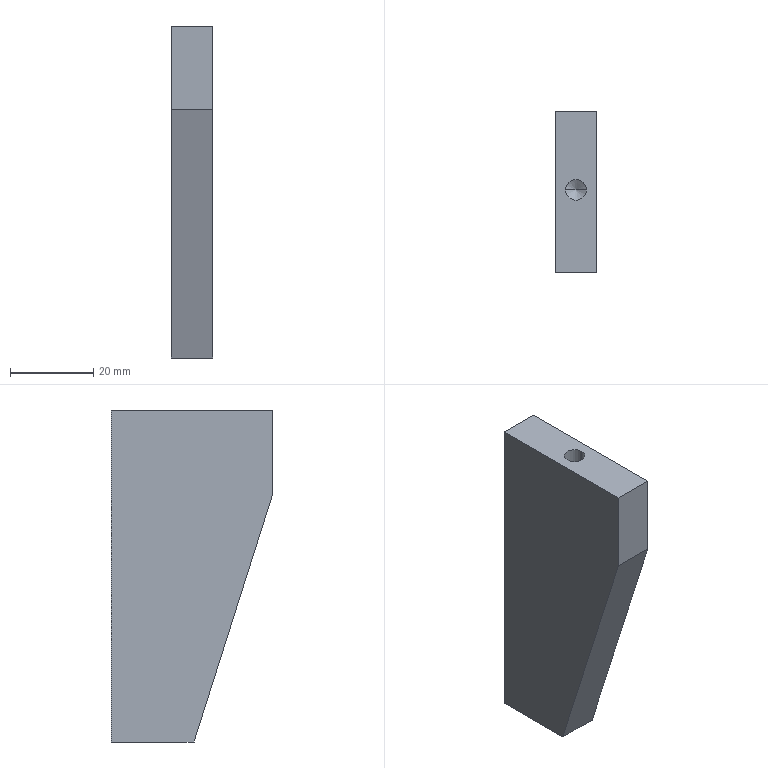Component | SolidWorks | 75-02-19StirringMotorSupportPlate-1 | 1 solid | 19 faces | box 10 x 39 x 80 mm | volume 24587 mm3 | plane 7 | cylinder 6 | cone 6 | commonest cylinder face diameters 5 x6 | material A3 Steel
build123d program:
from build123d import *

# Parameters (mm, degrees)
BOSS_EXTRUDE1_DEPTH   = 5
M6_TAPPED_HOLE1_D     = 5
M6_TAPPED_HOLE1_DEPTH = 15
M6_TAPPED_HOLE1_TIP   = 1.502
M6_TAPPED_HOLE2_D     = 5
M6_TAPPED_HOLE2_DEPTH = 15
M6_TAPPED_HOLE2_TIP   = 1.502


with BuildPart() as part:
    # Sketch1 → Boss-Extrude1 (new, symmetric)
    with BuildSketch(Plane.XY):
        Polygon((0, 39), (0, 0), (80, 0), (80, 20), (20, 39), align=None)
    extrude(amount=BOSS_EXTRUDE1_DEPTH, both=True)

    # M6 Tapped Hole1
    with Locations(Plane(origin=(60, 0, 0), x_dir=(0, 0, -1), z_dir=(0, -1, 0))):
        with Locations((0, 0), (0, -40)):
            Hole(M6_TAPPED_HOLE1_D / 2, depth=M6_TAPPED_HOLE1_DEPTH)
            with Locations((0, 0, -(M6_TAPPED_HOLE1_DEPTH + M6_TAPPED_HOLE1_TIP / 2))):  # 118° drill point
                Cone(0, M6_TAPPED_HOLE1_D / 2, M6_TAPPED_HOLE1_TIP, mode=Mode.SUBTRACT)

    # M6 Tapped Hole2
    with Locations(Plane(origin=(0, 19, 0), x_dir=(0, -1, 0), z_dir=(-1, 0, 0))):
        with Locations((0, 0)):
            Hole(M6_TAPPED_HOLE2_D / 2, depth=M6_TAPPED_HOLE2_DEPTH)
            with Locations((0, 0, -(M6_TAPPED_HOLE2_DEPTH + M6_TAPPED_HOLE2_TIP / 2))):  # 118° drill point
                Cone(0, M6_TAPPED_HOLE2_D / 2, M6_TAPPED_HOLE2_TIP, mode=Mode.SUBTRACT)


solid = part.part

# Placed as in the assembly
solid = solid.moved(Location((22.2, 105.857, 2.75), (180, -90, 0)))
STEP:
#1=COLOUR_RGB('',0.7922,0.8196,0.9333);
#2=FILL_AREA_STYLE_COLOUR('',#1);
#3=FILL_AREA_STYLE('',(#2));
#4=SURFACE_STYLE_FILL_AREA(#3);
#5=SURFACE_SIDE_STYLE('',(#4));
#6=SURFACE_STYLE_USAGE(.BOTH.,#5);
#7=PRESENTATION_STYLE_ASSIGNMENT((#6));
#8=CARTESIAN_POINT('',(0.9724,3.42,-0.4823));
#9=VERTEX_POINT('',#8);
#10=CARTESIAN_POINT('',(0.7756,3.42,-0.4823));
#11=VERTEX_POINT('',#10);
#12=CARTESIAN_POINT('',(0.874,3.42,-0.4823));
#13=DIRECTION('',(0.,-0.,1.));
#14=DIRECTION('',(-1.,0.,0.));
#15=AXIS2_PLACEMENT_3D('',#12,#13,#14);
#16=CIRCLE('',#15,0.09843);
#17=EDGE_CURVE('',#9,#11,#16,.T.);
#18=ORIENTED_EDGE('',*,*,#17,.F.);
#19=CARTESIAN_POINT('',(0.9724,3.42,0.1083));
#20=VERTEX_POINT('',#19);
#21=CARTESIAN_POINT('',(0.9724,3.42,0.1083));
#22=DIRECTION('',(0.,-0.,1.));
#23=VECTOR('',#22,39.37);
#24=LINE('',#21,#23);
#25=EDGE_CURVE('',#9,#20,#24,.T.);
#26=ORIENTED_EDGE('',*,*,#25,.T.);
#27=CARTESIAN_POINT('',(0.7756,3.42,0.1083));
#28=VERTEX_POINT('',#27);
#29=CARTESIAN_POINT('',(0.874,3.42,0.1083));
#30=DIRECTION('',(0.,-0.,1.));
#31=DIRECTION('',(-1.,0.,0.));
#32=AXIS2_PLACEMENT_3D('',#29,#30,#31);
#33=CIRCLE('',#32,0.09843);
#34=EDGE_CURVE('',#20,#28,#33,.T.);
#35=ORIENTED_EDGE('',*,*,#34,.T.);
#36=CARTESIAN_POINT('',(0.7756,3.42,0.1083));
#37=DIRECTION('',(0.,-0.,1.));
#38=VECTOR('',#37,39.37);
#39=LINE('',#36,#38);
#40=EDGE_CURVE('',#11,#28,#39,.T.);
#41=ORIENTED_EDGE('',*,*,#40,.F.);
#42=EDGE_LOOP('',(#18,#26,#35,#41));
#43=FACE_OUTER_BOUND('',#42,.T.);
#44=CARTESIAN_POINT('',(0.874,3.42,0.1083));
#45=DIRECTION('',(0.,-0.,1.));
#46=DIRECTION('',(-1.,0.,0.));
#47=AXIS2_PLACEMENT_3D('',#44,#45,#46);
#48=CYLINDRICAL_SURFACE('',#47,0.09843);
#49=ADVANCED_FACE('',(#43),#48,.F.);
#50=CARTESIAN_POINT('',(0.874,3.42,-0.5414));
#51=VERTEX_POINT('',#50);
#52=CARTESIAN_POINT('',(0.7756,3.42,-0.4823));
#53=DIRECTION('',(-0.8572,0.,0.515));
#54=VECTOR('',#53,39.37);
#55=LINE('',#52,#54);
#56=EDGE_CURVE('',#51,#11,#55,.T.);
#57=ORIENTED_EDGE('',*,*,#56,.F.);
#58=CARTESIAN_POINT('',(0.9724,3.42,-0.4823));
#59=DIRECTION('',(0.8572,-0.,0.515));
#60=VECTOR('',#59,39.37);
#61=LINE('',#58,#60);
#62=EDGE_CURVE('',#51,#9,#61,.T.);
#63=ORIENTED_EDGE('',*,*,#62,.T.);
#64=ORIENTED_EDGE('',*,*,#17,.T.);
#65=EDGE_LOOP('',(#57,#63,#64));
#66=FACE_OUTER_BOUND('',#65,.T.);
#67=CARTESIAN_POINT('',(0.874,3.42,-0.4823));
#68=DIRECTION('',(0.,-0.,1.));
#69=DIRECTION('',(-1.,0.,0.));
#70=AXIS2_PLACEMENT_3D('',#67,#68,#69);
#71=CONICAL_SURFACE('',#70,0.09843,1.03);
#72=ADVANCED_FACE('',(#66),#71,.F.);
#73=CARTESIAN_POINT('',(0.7756,3.577,-2.254));
#74=VERTEX_POINT('',#73);
#75=CARTESIAN_POINT('',(0.9724,3.577,-2.254));
#76=VERTEX_POINT('',#75);
#77=CARTESIAN_POINT('',(0.874,3.577,-2.254));
#78=DIRECTION('',(0.,1.,0.));
#79=DIRECTION('',(1.,0.,0.));
#80=AXIS2_PLACEMENT_3D('',#77,#78,#79);
#81=CIRCLE('',#80,0.09843);
#82=EDGE_CURVE('',#74,#76,#81,.T.);
#83=ORIENTED_EDGE('',*,*,#82,.F.);
#84=CARTESIAN_POINT('',(0.7756,4.168,-2.254));
#85=VERTEX_POINT('',#84);
#86=CARTESIAN_POINT('',(0.7756,4.168,-2.254));
#87=DIRECTION('',(0.,1.,0.));
#88=VECTOR('',#87,39.37);
#89=LINE('',#86,#88);
#90=EDGE_CURVE('',#74,#85,#89,.T.);
#91=ORIENTED_EDGE('',*,*,#90,.T.);
#92=CARTESIAN_POINT('',(0.9724,4.168,-2.254));
#93=VERTEX_POINT('',#92);
#94=CARTESIAN_POINT('',(0.874,4.168,-2.254));
#95=DIRECTION('',(0.,1.,0.));
#96=DIRECTION('',(1.,0.,0.));
#97=AXIS2_PLACEMENT_3D('',#94,#95,#96);
#98=CIRCLE('',#97,0.09843);
#99=EDGE_CURVE('',#85,#93,#98,.T.);
#100=ORIENTED_EDGE('',*,*,#99,.T.);
#101=CARTESIAN_POINT('',(0.9724,4.168,-2.254));
#102=DIRECTION('',(0.,1.,0.));
#103=VECTOR('',#102,39.37);
#104=LINE('',#101,#103);
#105=EDGE_CURVE('',#76,#93,#104,.T.);
#106=ORIENTED_EDGE('',*,*,#105,.F.);
#107=EDGE_LOOP('',(#83,#91,#100,#106));
#108=FACE_OUTER_BOUND('',#107,.T.);
#109=CARTESIAN_POINT('',(0.874,4.168,-2.254));
#110=DIRECTION('',(0.,1.,0.));
#111=DIRECTION('',(1.,0.,0.));
#112=AXIS2_PLACEMENT_3D('',#109,#110,#111);
#113=CYLINDRICAL_SURFACE('',#112,0.09843);
#114=ADVANCED_FACE('',(#108),#113,.F.);
#115=CARTESIAN_POINT('',(0.874,3.518,-2.254));
#116=VERTEX_POINT('',#115);
#117=CARTESIAN_POINT('',(0.9724,3.577,-2.254));
#118=DIRECTION('',(0.8572,0.515,-0.));
#119=VECTOR('',#118,39.37);
#120=LINE('',#117,#119);
#121=EDGE_CURVE('',#116,#76,#120,.T.);
#122=ORIENTED_EDGE('',*,*,#121,.F.);
#123=CARTESIAN_POINT('',(0.7756,3.577,-2.254));
#124=DIRECTION('',(-0.8572,0.515,0.));
#125=VECTOR('',#124,39.37);
#126=LINE('',#123,#125);
#127=EDGE_CURVE('',#116,#74,#126,.T.);
#128=ORIENTED_EDGE('',*,*,#127,.T.);
#129=ORIENTED_EDGE('',*,*,#82,.T.);
#130=EDGE_LOOP('',(#122,#128,#129));
#131=FACE_OUTER_BOUND('',#130,.T.);
#132=CARTESIAN_POINT('',(0.874,3.577,-2.254));
#133=DIRECTION('',(0.,1.,0.));
#134=DIRECTION('',(1.,0.,0.));
#135=AXIS2_PLACEMENT_3D('',#132,#133,#134);
#136=CONICAL_SURFACE('',#135,0.09843,1.03);
#137=ADVANCED_FACE('',(#131),#136,.F.);
#138=CARTESIAN_POINT('',(0.7756,3.577,-0.6791));
#139=VERTEX_POINT('',#138);
#140=CARTESIAN_POINT('',(0.9724,3.577,-0.6791));
#141=VERTEX_POINT('',#140);
#142=CARTESIAN_POINT('',(0.874,3.577,-0.6791));
#143=DIRECTION('',(0.,1.,0.));
#144=DIRECTION('',(1.,0.,0.));
#145=AXIS2_PLACEMENT_3D('',#142,#143,#144);
#146=CIRCLE('',#145,0.09843);
#147=EDGE_CURVE('',#139,#141,#146,.T.);
#148=ORIENTED_EDGE('',*,*,#147,.F.);
#149=CARTESIAN_POINT('',(0.7756,4.168,-0.6791));
#150=VERTEX_POINT('',#149);
#151=CARTESIAN_POINT('',(0.7756,4.168,-0.6791));
#152=DIRECTION('',(0.,1.,0.));
#153=VECTOR('',#152,39.37);
#154=LINE('',#151,#153);
#155=EDGE_CURVE('',#139,#150,#154,.T.);
#156=ORIENTED_EDGE('',*,*,#155,.T.);
#157=CARTESIAN_POINT('',(0.9724,4.168,-0.6791));
#158=VERTEX_POINT('',#157);
#159=CARTESIAN_POINT('',(0.874,4.168,-0.6791));
#160=DIRECTION('',(0.,1.,0.));
#161=DIRECTION('',(1.,0.,0.));
#162=AXIS2_PLACEMENT_3D('',#159,#160,#161);
#163=CIRCLE('',#162,0.09843);
#164=EDGE_CURVE('',#150,#158,#163,.T.);
#165=ORIENTED_EDGE('',*,*,#164,.T.);
#166=CARTESIAN_POINT('',(0.9724,4.168,-0.6791));
#167=DIRECTION('',(0.,1.,0.));
#168=VECTOR('',#167,39.37);
#169=LINE('',#166,#168);
#170=EDGE_CURVE('',#141,#158,#169,.T.);
#171=ORIENTED_EDGE('',*,*,#170,.F.);
#172=EDGE_LOOP('',(#148,#156,#165,#171));
#173=FACE_OUTER_BOUND('',#172,.T.);
#174=CARTESIAN_POINT('',(0.874,4.168,-0.6791));
#175=DIRECTION('',(0.,1.,0.));
#176=DIRECTION('',(1.,0.,0.));
#177=AXIS2_PLACEMENT_3D('',#174,#175,#176);
#178=CYLINDRICAL_SURFACE('',#177,0.09843);
#179=ADVANCED_FACE('',(#173),#178,.F.);
#180=CARTESIAN_POINT('',(0.874,3.518,-0.6791));
#181=VERTEX_POINT('',#180);
#182=CARTESIAN_POINT('',(0.9724,3.577,-0.6791));
#183=DIRECTION('',(0.8572,0.515,-0.));
#184=VECTOR('',#183,39.37);
#185=LINE('',#182,#184);
#186=EDGE_CURVE('',#181,#141,#185,.T.);
#187=ORIENTED_EDGE('',*,*,#186,.F.);
#188=CARTESIAN_POINT('',(0.7756,3.577,-0.6791));
#189=DIRECTION('',(-0.8572,0.515,0.));
#190=VECTOR('',#189,39.37);
#191=LINE('',#188,#190);
#192=EDGE_CURVE('',#181,#139,#191,.T.);
#193=ORIENTED_EDGE('',*,*,#192,.T.);
#194=ORIENTED_EDGE('',*,*,#147,.T.);
#195=EDGE_LOOP('',(#187,#193,#194));
#196=FACE_OUTER_BOUND('',#195,.T.);
#197=CARTESIAN_POINT('',(0.874,3.577,-0.6791));
#198=DIRECTION('',(0.,1.,0.));
#199=DIRECTION('',(1.,0.,0.));
#200=AXIS2_PLACEMENT_3D('',#197,#198,#199);
#201=CONICAL_SURFACE('',#200,0.09843,1.03);
#202=ADVANCED_FACE('',(#196),#201,.F.);
#203=CARTESIAN_POINT('',(1.071,2.632,-0.6791));
#204=VERTEX_POINT('',#203);
#205=CARTESIAN_POINT('',(1.071,2.632,0.1083));
#206=VERTEX_POINT('',#205);
#207=CARTESIAN_POINT('',(1.071,2.632,-0.6791));
#208=DIRECTION('',(0.,-0.,1.));
#209=VECTOR('',#208,39.37);
#210=LINE('',#207,#209);
#211=EDGE_CURVE('',#204,#206,#210,.T.);
#212=ORIENTED_EDGE('',*,*,#211,.T.);
#213=CARTESIAN_POINT('',(0.6772,2.632,0.1083));
#214=VERTEX_POINT('',#213);
#215=CARTESIAN_POINT('',(0.6772,2.632,0.1083));
#216=DIRECTION('',(1.,-0.,-0.));
#217=VECTOR('',#216,39.37);
#218=LINE('',#215,#217);
#219=EDGE_CURVE('',#214,#206,#218,.T.);
#220=ORIENTED_EDGE('',*,*,#219,.F.);
#221=CARTESIAN_POINT('',(0.6772,2.632,-0.6791));
#222=VERTEX_POINT('',#221);
#223=CARTESIAN_POINT('',(0.6772,2.632,-0.6791));
#224=DIRECTION('',(0.,-0.,1.));
#225=VECTOR('',#224,39.37);
#226=LINE('',#223,#225);
#227=EDGE_CURVE('',#222,#214,#226,.T.);
#228=ORIENTED_EDGE('',*,*,#227,.F.);
#229=CARTESIAN_POINT('',(0.6772,2.632,-0.6791));
#230=DIRECTION('',(1.,-0.,-0.));
#231=VECTOR('',#230,39.37);
#232=LINE('',#229,#231);
#233=EDGE_CURVE('',#222,#204,#232,.T.);
#234=ORIENTED_EDGE('',*,*,#233,.T.);
#235=EDGE_LOOP('',(#212,#220,#228,#234));
#236=FACE_OUTER_BOUND('',#235,.T.);
#237=CARTESIAN_POINT('',(0.6772,2.632,-0.6791));
#238=DIRECTION('',(0.,1.,0.));
#239=DIRECTION('',(1.,-0.,-0.));
#240=AXIS2_PLACEMENT_3D('',#237,#238,#239);
#241=PLANE('',#240);
#242=ADVANCED_FACE('',(#236),#241,.F.);
#243=CARTESIAN_POINT('',(0.874,3.42,0.1083));
#244=DIRECTION('',(0.,-0.,1.));
#245=DIRECTION('',(-1.,0.,0.));
#246=AXIS2_PLACEMENT_3D('',#243,#244,#245);
#247=CIRCLE('',#246,0.09843);
#248=EDGE_CURVE('',#28,#20,#247,.T.);
#249=ORIENTED_EDGE('',*,*,#248,.F.);
#250=ORIENTED_EDGE('',*,*,#34,.F.);
#251=EDGE_LOOP('',(#249,#250));
#252=FACE_BOUND('',#251,.T.);
#253=CARTESIAN_POINT('',(1.071,4.168,0.1083));
#254=VERTEX_POINT('',#253);
#255=CARTESIAN_POINT('',(1.071,2.632,0.1083));
#256=DIRECTION('',(0.,1.,0.));
#257=VECTOR('',#256,39.37);
#258=LINE('',#255,#257);
#259=EDGE_CURVE('',#206,#254,#258,.T.);
#260=ORIENTED_EDGE('',*,*,#259,.T.);
#261=CARTESIAN_POINT('',(0.6772,4.168,0.1083));
#262=VERTEX_POINT('',#261);
#263=CARTESIAN_POINT('',(0.6772,4.168,0.1083));
#264=DIRECTION('',(1.,-0.,-0.));
#265=VECTOR('',#264,39.37);
#266=LINE('',#263,#265);
#267=EDGE_CURVE('',#262,#254,#266,.T.);
#268=ORIENTED_EDGE('',*,*,#267,.F.);
#269=CARTESIAN_POINT('',(0.6772,2.632,0.1083));
#270=DIRECTION('',(0.,1.,0.));
#271=VECTOR('',#270,39.37);
#272=LINE('',#269,#271);
#273=EDGE_CURVE('',#214,#262,#272,.T.);
#274=ORIENTED_EDGE('',*,*,#273,.F.);
#275=ORIENTED_EDGE('',*,*,#219,.T.);
#276=EDGE_LOOP('',(#260,#268,#274,#275));
#277=FACE_OUTER_BOUND('',#276,.T.);
#278=CARTESIAN_POINT('',(0.6772,2.632,0.1083));
#279=DIRECTION('',(-0.,0.,-1.));
#280=DIRECTION('',(-0.,-1.,-0.));
#281=AXIS2_PLACEMENT_3D('',#278,#279,#280);
#282=PLANE('',#281);
#283=ADVANCED_FACE('',(#252,#277),#282,.F.);
#284=CARTESIAN_POINT('',(0.874,4.168,-2.254));
#285=DIRECTION('',(0.,1.,0.));
#286=DIRECTION('',(1.,0.,0.));
#287=AXIS2_PLACEMENT_3D('',#284,#285,#286);
#288=CIRCLE('',#287,0.09843);
#289=EDGE_CURVE('',#93,#85,#288,.T.);
#290=ORIENTED_EDGE('',*,*,#289,.F.);
#291=ORIENTED_EDGE('',*,*,#99,.F.);
#292=EDGE_LOOP('',(#290,#291));
#293=FACE_BOUND('',#292,.T.);
#294=CARTESIAN_POINT('',(0.874,4.168,-0.6791));
#295=DIRECTION('',(0.,1.,0.));
#296=DIRECTION('',(1.,0.,0.));
#297=AXIS2_PLACEMENT_3D('',#294,#295,#296);
#298=CIRCLE('',#297,0.09843);
#299=EDGE_CURVE('',#158,#150,#298,.T.);
#300=ORIENTED_EDGE('',*,*,#299,.F.);
#301=ORIENTED_EDGE('',*,*,#164,.F.);
#302=EDGE_LOOP('',(#300,#301));
#303=FACE_BOUND('',#302,.T.);
#304=CARTESIAN_POINT('',(1.071,4.168,-3.041));
#305=VERTEX_POINT('',#304);
#306=CARTESIAN_POINT('',(1.071,4.168,0.1083));
#307=DIRECTION('',(-0.,0.,-1.));
#308=VECTOR('',#307,39.37);
#309=LINE('',#306,#308);
#310=EDGE_CURVE('',#254,#305,#309,.T.);
#311=ORIENTED_EDGE('',*,*,#310,.T.);
#312=CARTESIAN_POINT('',(0.6772,4.168,-3.041));
#313=VERTEX_POINT('',#312);
#314=CARTESIAN_POINT('',(0.6772,4.168,-3.041));
#315=DIRECTION('',(1.,-0.,-0.));
#316=VECTOR('',#315,39.37);
#317=LINE('',#314,#316);
#318=EDGE_CURVE('',#313,#305,#317,.T.);
#319=ORIENTED_EDGE('',*,*,#318,.F.);
#320=CARTESIAN_POINT('',(0.6772,4.168,0.1083));
#321=DIRECTION('',(-0.,0.,-1.));
#322=VECTOR('',#321,39.37);
#323=LINE('',#320,#322);
#324=EDGE_CURVE('',#262,#313,#323,.T.);
#325=ORIENTED_EDGE('',*,*,#324,.F.);
#326=ORIENTED_EDGE('',*,*,#267,.T.);
#327=EDGE_LOOP('',(#311,#319,#325,#326));
#328=FACE_OUTER_BOUND('',#327,.T.);
#329=CARTESIAN_POINT('',(0.6772,4.168,0.1083));
#330=DIRECTION('',(-0.,-1.,-0.));
#331=DIRECTION('',(-1.,0.,0.));
#332=AXIS2_PLACEMENT_3D('',#329,#330,#331);
#333=PLANE('',#332);
#334=ADVANCED_FACE('',(#293,#303,#328),#333,.F.);
#335=CARTESIAN_POINT('',(1.071,3.38,-3.041));
#336=VERTEX_POINT('',#335);
#337=CARTESIAN_POINT('',(1.071,4.168,-3.041));
#338=DIRECTION('',(-0.,-1.,-0.));
#339=VECTOR('',#338,39.37);
#340=LINE('',#337,#339);
#341=EDGE_CURVE('',#305,#336,#340,.T.);
#342=ORIENTED_EDGE('',*,*,#341,.T.);
#343=CARTESIAN_POINT('',(0.6772,3.38,-3.041));
#344=VERTEX_POINT('',#343);
#345=CARTESIAN_POINT('',(0.6772,3.38,-3.041));
#346=DIRECTION('',(1.,-0.,-0.));
#347=VECTOR('',#346,39.37);
#348=LINE('',#345,#347);
#349=EDGE_CURVE('',#344,#336,#348,.T.);
#350=ORIENTED_EDGE('',*,*,#349,.F.);
#351=CARTESIAN_POINT('',(0.6772,4.168,-3.041));
#352=DIRECTION('',(-0.,-1.,-0.));
#353=VECTOR('',#352,39.37);
#354=LINE('',#351,#353);
#355=EDGE_CURVE('',#313,#344,#354,.T.);
#356=ORIENTED_EDGE('',*,*,#355,.F.);
#357=ORIENTED_EDGE('',*,*,#318,.T.);
#358=EDGE_LOOP('',(#342,#350,#356,#357));
#359=FACE_OUTER_BOUND('',#358,.T.);
#360=CARTESIAN_POINT('',(0.6772,4.168,-3.041));
#361=DIRECTION('',(0.,-0.,1.));
#362=DIRECTION('',(-1.,0.,0.));
#363=AXIS2_PLACEMENT_3D('',#360,#361,#362);
#364=PLANE('',#363);
#365=ADVANCED_FACE('',(#359),#364,.F.);
#366=CARTESIAN_POINT('',(1.071,3.38,-3.041));
#367=DIRECTION('',(0.,-0.3019,0.9533));
#368=VECTOR('',#367,39.37);
#369=LINE('',#366,#368);
#370=EDGE_CURVE('',#336,#204,#369,.T.);
#371=ORIENTED_EDGE('',*,*,#370,.T.);
#372=ORIENTED_EDGE('',*,*,#233,.F.);
#373=CARTESIAN_POINT('',(0.6772,3.38,-3.041));
#374=DIRECTION('',(0.,-0.3019,0.9533));
#375=VECTOR('',#374,39.37);
#376=LINE('',#373,#375);
#377=EDGE_CURVE('',#344,#222,#376,.T.);
#378=ORIENTED_EDGE('',*,*,#377,.F.);
#379=ORIENTED_EDGE('',*,*,#349,.T.);
#380=EDGE_LOOP('',(#371,#372,#378,#379));
#381=FACE_OUTER_BOUND('',#380,.T.);
#382=CARTESIAN_POINT('',(0.6772,3.38,-3.041));
#383=DIRECTION('',(0.,0.9533,0.3019));
#384=DIRECTION('',(-0.,0.3019,-0.9533));
#385=AXIS2_PLACEMENT_3D('',#382,#383,#384);
#386=PLANE('',#385);
#387=ADVANCED_FACE('',(#381),#386,.F.);
#388=ORIENTED_EDGE('',*,*,#227,.T.);
#389=ORIENTED_EDGE('',*,*,#273,.T.);
#390=ORIENTED_EDGE('',*,*,#324,.T.);
#391=ORIENTED_EDGE('',*,*,#355,.T.);
#392=ORIENTED_EDGE('',*,*,#377,.T.);
#393=EDGE_LOOP('',(#388,#389,#390,#391,#392));
#394=FACE_OUTER_BOUND('',#393,.T.);
#395=CARTESIAN_POINT('',(0.6772,4.168,0.1083));
#396=DIRECTION('',(-1.,0.,0.));
#397=DIRECTION('',(-0.,0.,-1.));
#398=AXIS2_PLACEMENT_3D('',#395,#396,#397);
#399=PLANE('',#398);
#400=ADVANCED_FACE('',(#394),#399,.T.);
#401=ORIENTED_EDGE('',*,*,#211,.F.);
#402=ORIENTED_EDGE('',*,*,#370,.F.);
#403=ORIENTED_EDGE('',*,*,#341,.F.);
#404=ORIENTED_EDGE('',*,*,#310,.F.);
#405=ORIENTED_EDGE('',*,*,#259,.F.);
#406=EDGE_LOOP('',(#401,#402,#403,#404,#405));
#407=FACE_OUTER_BOUND('',#406,.T.);
#408=CARTESIAN_POINT('',(1.071,4.168,0.1083));
#409=DIRECTION('',(-1.,0.,0.));
#410=DIRECTION('',(-0.,0.,-1.));
#411=AXIS2_PLACEMENT_3D('',#408,#409,#410);
#412=PLANE('',#411);
#413=ADVANCED_FACE('',(#407),#412,.F.);
#414=ORIENTED_EDGE('',*,*,#192,.F.);
#415=ORIENTED_EDGE('',*,*,#186,.T.);
#416=CARTESIAN_POINT('',(0.874,3.577,-0.6791));
#417=DIRECTION('',(0.,1.,0.));
#418=DIRECTION('',(1.,0.,0.));
#419=AXIS2_PLACEMENT_3D('',#416,#417,#418);
#420=CIRCLE('',#419,0.09843);
#421=EDGE_CURVE('',#141,#139,#420,.T.);
#422=ORIENTED_EDGE('',*,*,#421,.T.);
#423=EDGE_LOOP('',(#414,#415,#422));
#424=FACE_OUTER_BOUND('',#423,.T.);
#425=CARTESIAN_POINT('',(0.874,3.577,-0.6791));
#426=DIRECTION('',(0.,1.,0.));
#427=DIRECTION('',(1.,0.,0.));
#428=AXIS2_PLACEMENT_3D('',#425,#426,#427);
#429=CONICAL_SURFACE('',#428,0.09843,1.03);
#430=ADVANCED_FACE('',(#424),#429,.F.);
#431=ORIENTED_EDGE('',*,*,#155,.F.);
#432=ORIENTED_EDGE('',*,*,#421,.F.);
#433=ORIENTED_EDGE('',*,*,#170,.T.);
#434=ORIENTED_EDGE('',*,*,#299,.T.);
#435=EDGE_LOOP('',(#431,#432,#433,#434));
#436=FACE_OUTER_BOUND('',#435,.T.);
#437=CARTESIAN_POINT('',(0.874,4.168,-0.6791));
#438=DIRECTION('',(0.,1.,0.));
#439=DIRECTION('',(1.,0.,0.));
#440=AXIS2_PLACEMENT_3D('',#437,#438,#439);
#441=CYLINDRICAL_SURFACE('',#440,0.09843);
#442=ADVANCED_FACE('',(#436),#441,.F.);
#443=ORIENTED_EDGE('',*,*,#127,.F.);
#444=ORIENTED_EDGE('',*,*,#121,.T.);
#445=CARTESIAN_POINT('',(0.874,3.577,-2.254));
#446=DIRECTION('',(0.,1.,0.));
#447=DIRECTION('',(1.,0.,0.));
#448=AXIS2_PLACEMENT_3D('',#445,#446,#447);
#449=CIRCLE('',#448,0.09843);
#450=EDGE_CURVE('',#76,#74,#449,.T.);
#451=ORIENTED_EDGE('',*,*,#450,.T.);
#452=EDGE_LOOP('',(#443,#444,#451));
#453=FACE_OUTER_BOUND('',#452,.T.);
#454=CARTESIAN_POINT('',(0.874,3.577,-2.254));
#455=DIRECTION('',(0.,1.,0.));
#456=DIRECTION('',(1.,0.,0.));
#457=AXIS2_PLACEMENT_3D('',#454,#455,#456);
#458=CONICAL_SURFACE('',#457,0.09843,1.03);
#459=ADVANCED_FACE('',(#453),#458,.F.);
#460=ORIENTED_EDGE('',*,*,#90,.F.);
#461=ORIENTED_EDGE('',*,*,#450,.F.);
#462=ORIENTED_EDGE('',*,*,#105,.T.);
#463=ORIENTED_EDGE('',*,*,#289,.T.);
#464=EDGE_LOOP('',(#460,#461,#462,#463));
#465=FACE_OUTER_BOUND('',#464,.T.);
#466=CARTESIAN_POINT('',(0.874,4.168,-2.254));
#467=DIRECTION('',(0.,1.,0.));
#468=DIRECTION('',(1.,0.,0.));
#469=AXIS2_PLACEMENT_3D('',#466,#467,#468);
#470=CYLINDRICAL_SURFACE('',#469,0.09843);
#471=ADVANCED_FACE('',(#465),#470,.F.);
#472=ORIENTED_EDGE('',*,*,#62,.F.);
#473=ORIENTED_EDGE('',*,*,#56,.T.);
#474=CARTESIAN_POINT('',(0.874,3.42,-0.4823));
#475=DIRECTION('',(0.,-0.,1.));
#476=DIRECTION('',(-1.,0.,0.));
#477=AXIS2_PLACEMENT_3D('',#474,#475,#476);
#478=CIRCLE('',#477,0.09843);
#479=EDGE_CURVE('',#11,#9,#478,.T.);
#480=ORIENTED_EDGE('',*,*,#479,.T.);
#481=EDGE_LOOP('',(#472,#473,#480));
#482=FACE_OUTER_BOUND('',#481,.T.);
#483=CARTESIAN_POINT('',(0.874,3.42,-0.4823));
#484=DIRECTION('',(0.,-0.,1.));
#485=DIRECTION('',(-1.,0.,0.));
#486=AXIS2_PLACEMENT_3D('',#483,#484,#485);
#487=CONICAL_SURFACE('',#486,0.09843,1.03);
#488=ADVANCED_FACE('',(#482),#487,.F.);
#489=ORIENTED_EDGE('',*,*,#25,.F.);
#490=ORIENTED_EDGE('',*,*,#479,.F.);
#491=ORIENTED_EDGE('',*,*,#40,.T.);
#492=ORIENTED_EDGE('',*,*,#248,.T.);
#493=EDGE_LOOP('',(#489,#490,#491,#492));
#494=FACE_OUTER_BOUND('',#493,.T.);
#495=CARTESIAN_POINT('',(0.874,3.42,0.1083));
#496=DIRECTION('',(0.,-0.,1.));
#497=DIRECTION('',(-1.,0.,0.));
#498=AXIS2_PLACEMENT_3D('',#495,#496,#497);
#499=CYLINDRICAL_SURFACE('',#498,0.09843);
#500=ADVANCED_FACE('',(#494),#499,.F.);
#501=CLOSED_SHELL('',(#49,#72,#114,#137,#179,#202,#242,#283,#334,#365,#387,#400,#413,#430,#442,#459,#471,#488,#500));
#502=MANIFOLD_SOLID_BREP('',#501);
#503=STYLED_ITEM('',(#7),#502);
#504=(LENGTH_UNIT()NAMED_UNIT(*)SI_UNIT($,.METRE.));
#505=LENGTH_MEASURE_WITH_UNIT(LENGTH_MEASURE(0.0254),#504);
#506=DIMENSIONAL_EXPONENTS(1.,0.,0.,0.,0.,0.,0.);
#507=(CONVERSION_BASED_UNIT('',#505)LENGTH_UNIT()NAMED_UNIT(#506));
#508=UNCERTAINTY_MEASURE_WITH_UNIT(LENGTH_MEASURE(0.00001),#507,'','');
#509=(NAMED_UNIT(*)PLANE_ANGLE_UNIT()SI_UNIT($,.RADIAN.));
#510=(NAMED_UNIT(*)SI_UNIT($,.STERADIAN.)SOLID_ANGLE_UNIT());
#511=(GEOMETRIC_REPRESENTATION_CONTEXT(3)GLOBAL_UNCERTAINTY_ASSIGNED_CONTEXT((#508))GLOBAL_UNIT_ASSIGNED_CONTEXT((#507,#509,#510))REPRESENTATION_CONTEXT('',''));
#512=MECHANICAL_DESIGN_GEOMETRIC_PRESENTATION_REPRESENTATION('',(#503),#511);
#513=PRESENTATION_LAYER_ASSIGNMENT('','',(#503));
#514=CARTESIAN_POINT('',(0.,0.,0.));
#515=DIRECTION('',(0.,0.,1.));
#516=DIRECTION('',(1.,0.,0.));
#517=AXIS2_PLACEMENT_3D('',#514,#515,#516);
#518=(LENGTH_UNIT()NAMED_UNIT(*)SI_UNIT($,.METRE.));
#519=LENGTH_MEASURE_WITH_UNIT(LENGTH_MEASURE(0.0254),#518);
#520=DIMENSIONAL_EXPONENTS(1.,0.,0.,0.,0.,0.,0.);
#521=(CONVERSION_BASED_UNIT('',#519)LENGTH_UNIT()NAMED_UNIT(#520));
#522=UNCERTAINTY_MEASURE_WITH_UNIT(LENGTH_MEASURE(0.00001),#521,'','');
#523=(NAMED_UNIT(*)PLANE_ANGLE_UNIT()SI_UNIT($,.RADIAN.));
#524=(NAMED_UNIT(*)SI_UNIT($,.STERADIAN.)SOLID_ANGLE_UNIT());
#525=(GEOMETRIC_REPRESENTATION_CONTEXT(3)GLOBAL_UNCERTAINTY_ASSIGNED_CONTEXT((#522))GLOBAL_UNIT_ASSIGNED_CONTEXT((#521,#523,#524))REPRESENTATION_CONTEXT('',''));
#526=ADVANCED_BREP_SHAPE_REPRESENTATION('',(#502,#517),#525);